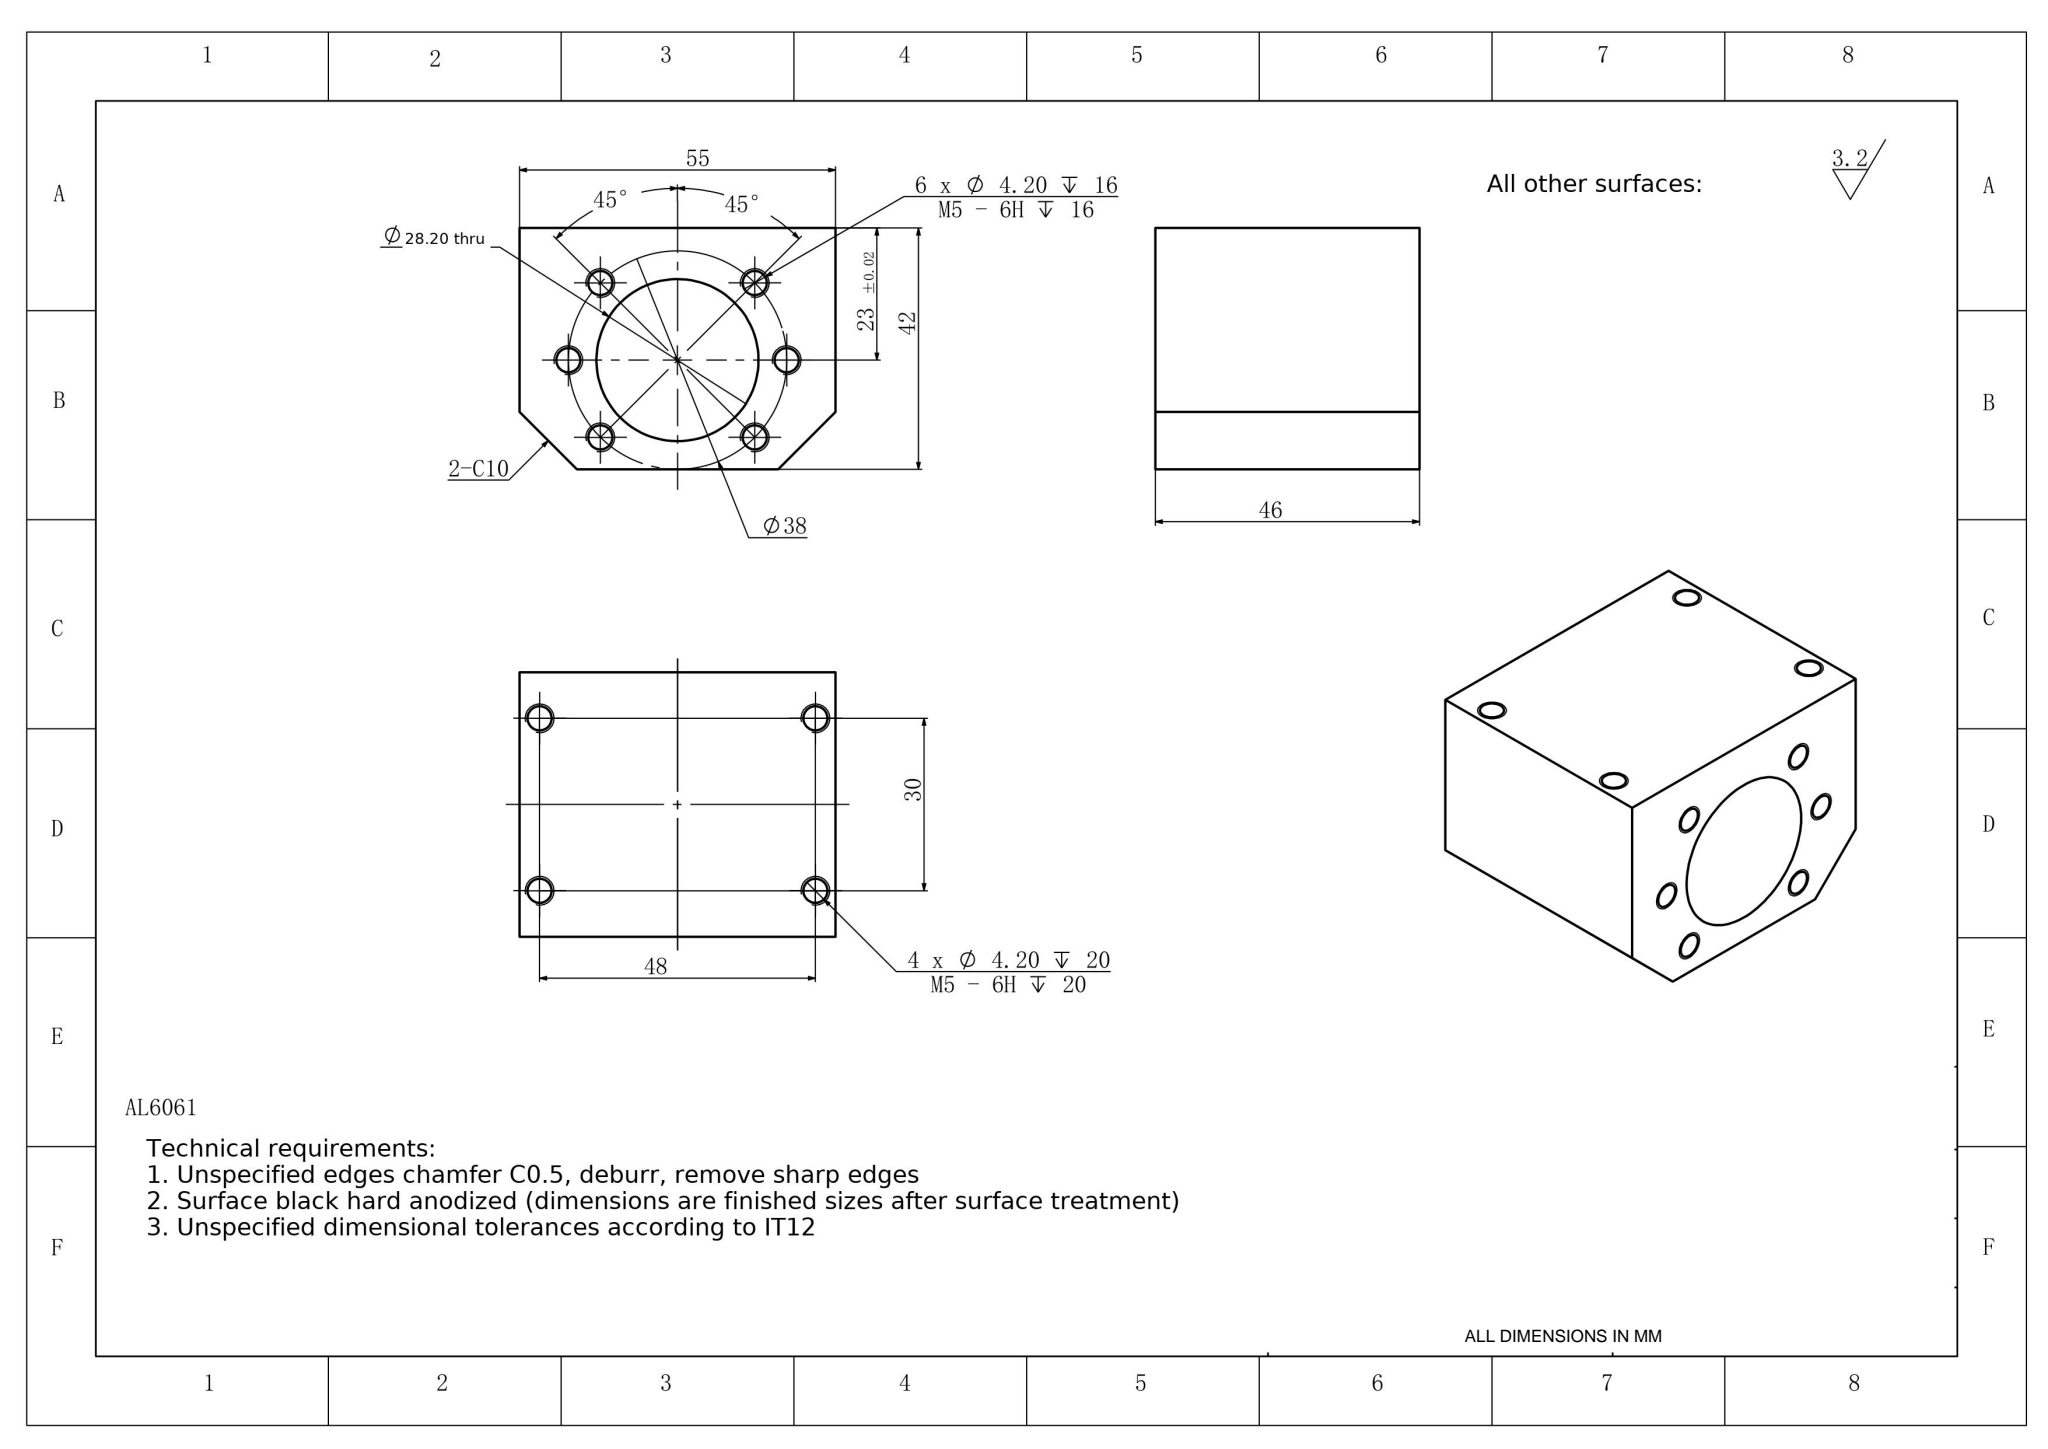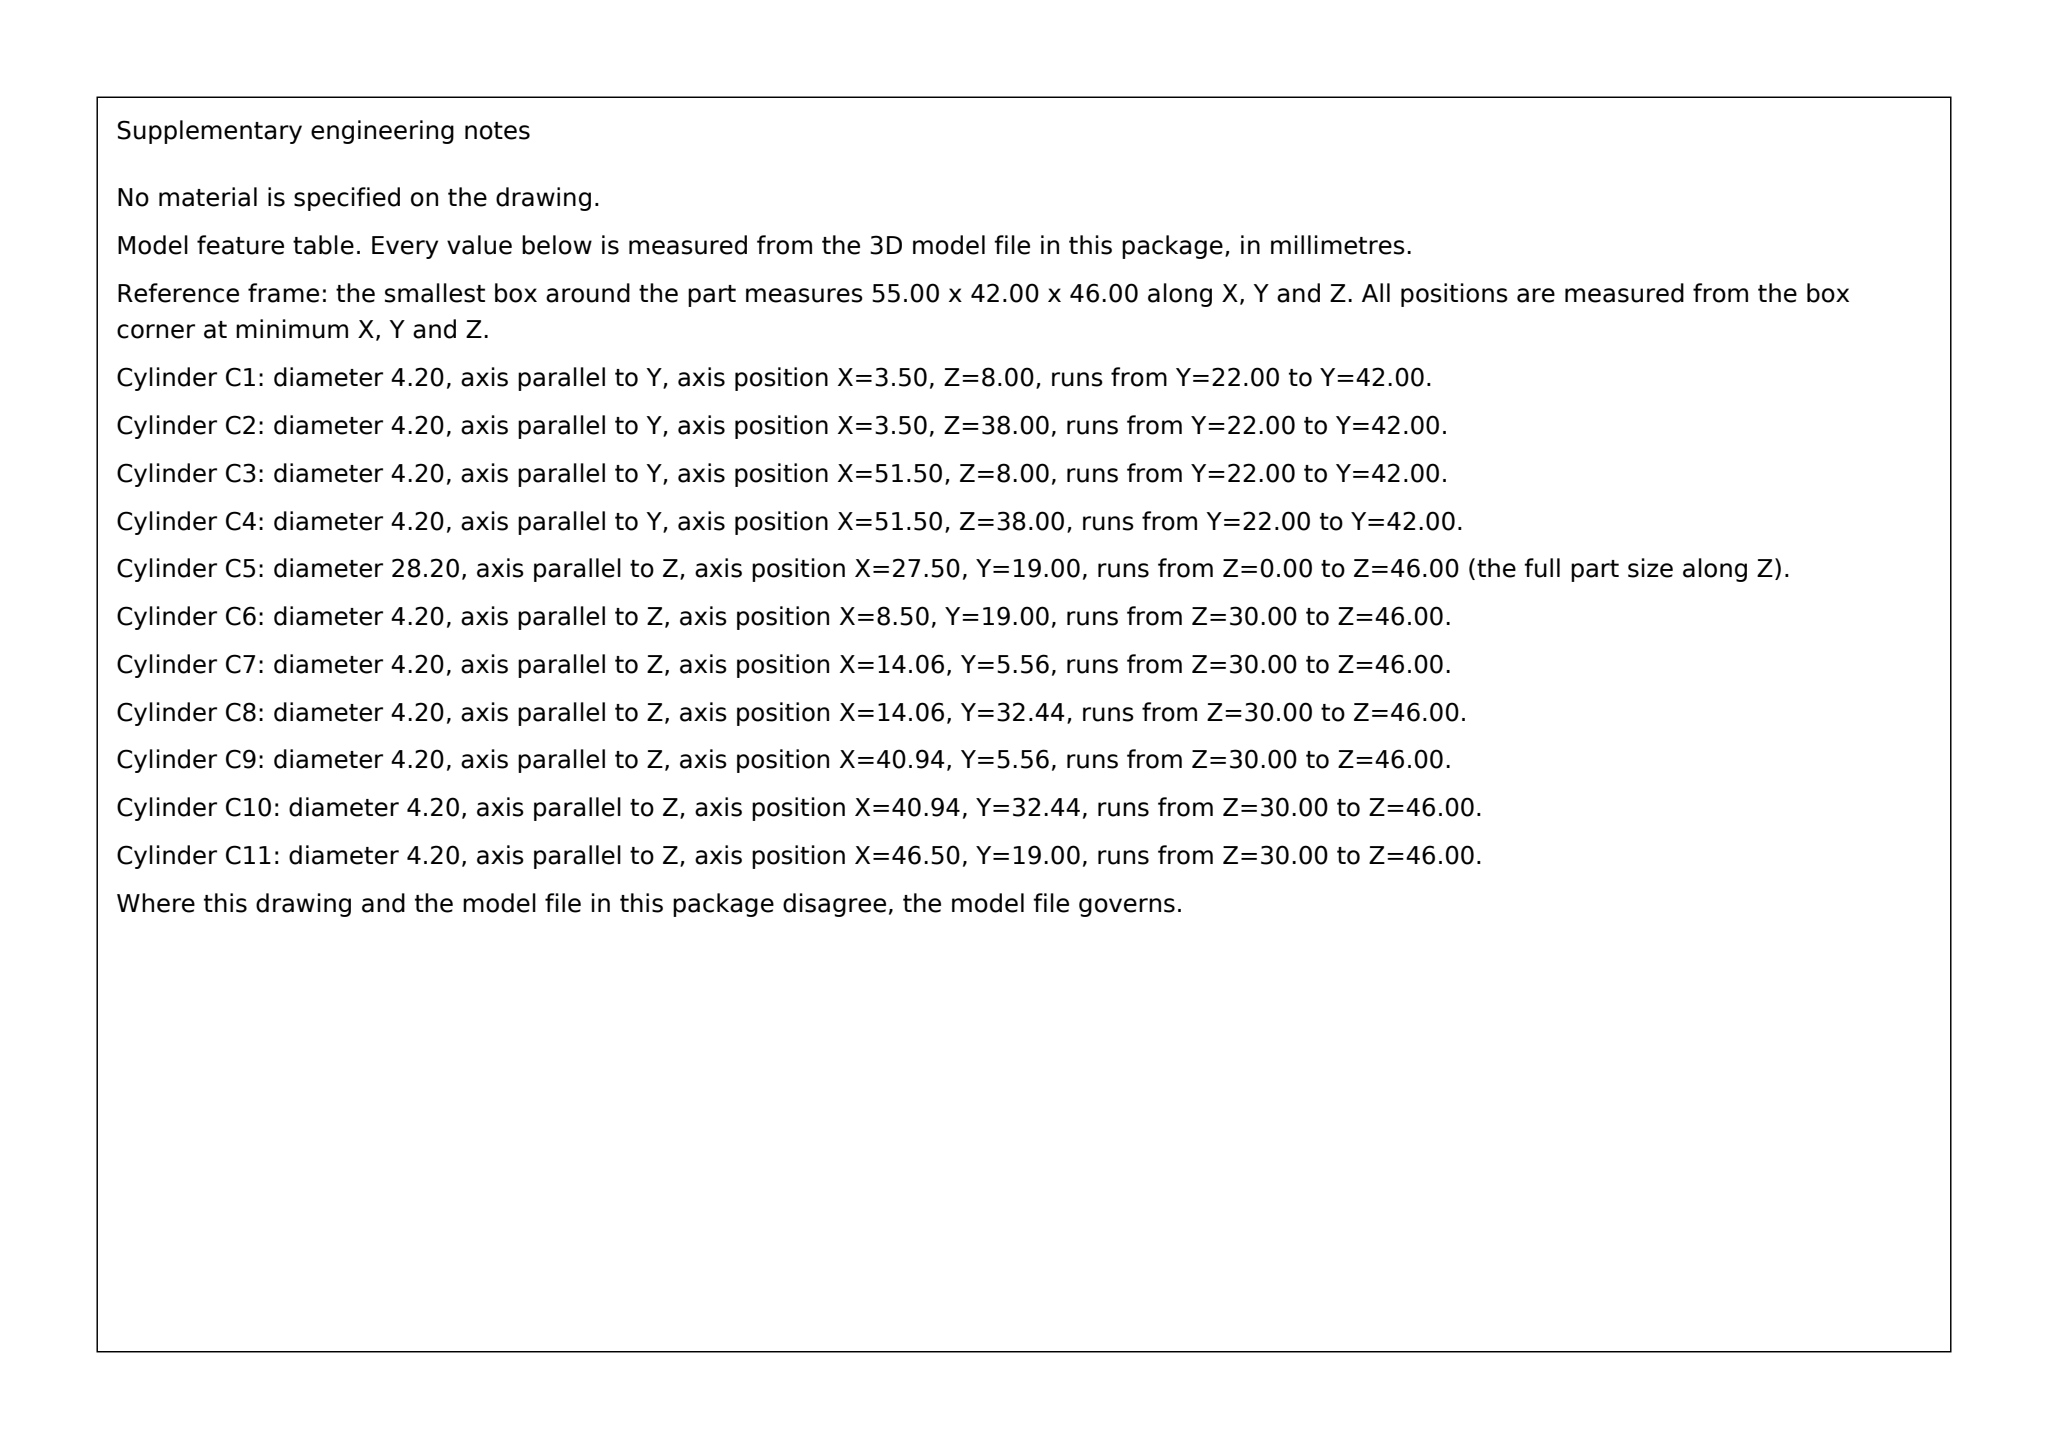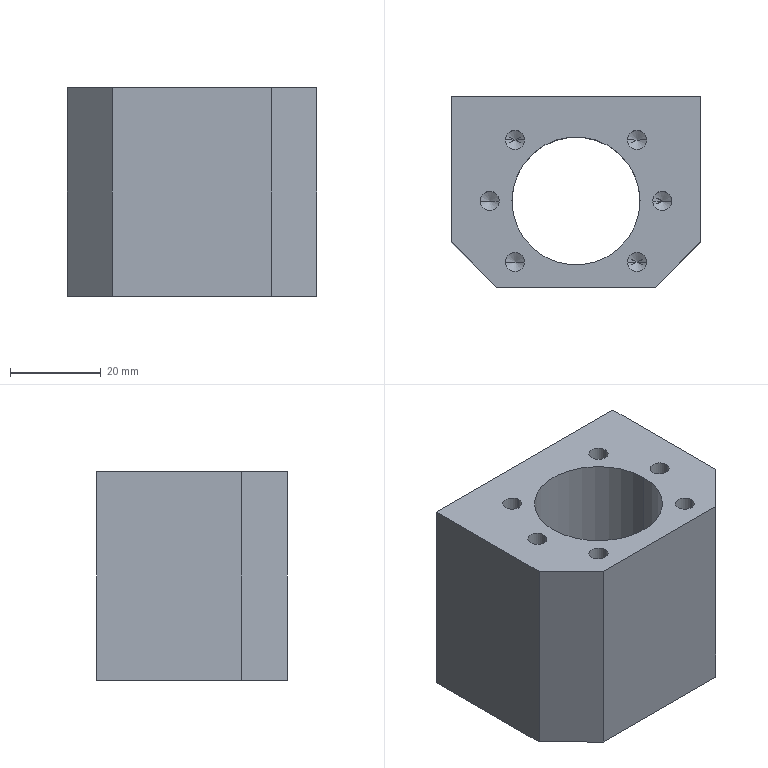Part | SolidWorks | mm | material AL6061 | 1 solid | 50 faces | box 55 x 42 x 46 mm | volume 70433 mm3 | cylinder 22 | cone 20 | plane 8 | commonest cylinder face diameters 4.2 x20 28.2 x2
build123d program:
from build123d import *

# Parameters (mm, degrees)
SKETCH1_W             = 55
SKETCH1_H             = 42
SKETCH1_R             = 14.1
EXTRUDE1_DEPTH        = 46
M5_TAPPED_HOLE3_D     = 4.2
M5_TAPPED_HOLE3_DEPTH = 16
M5_TAPPED_HOLE3_TIP   = 1.262
M5_TAPPED_HOLE4_D     = 4.2
M5_TAPPED_HOLE4_DEPTH = 20
M5_TAPPED_HOLE4_TIP   = 1.262
CHAMFER1_SIZE         = 10


with BuildPart() as part:
    # Sketch1 → Extrude1 (new body)
    with BuildSketch(Plane.XY):
        with Locations((27.5, 21)):
            Rectangle(SKETCH1_W, SKETCH1_H)
        with Locations((27.5, 19)):
            Circle(SKETCH1_R, mode=Mode.SUBTRACT)
    extrude(amount=EXTRUDE1_DEPTH)

    # M5 Tapped Hole3
    with Locations(Plane.XY.offset(46)):
        with Locations((14.065, 32.435), (8.5, 19), (14.065, 5.565), (40.935, 32.435), (46.5, 19), (40.935, 5.565)):
            Hole(M5_TAPPED_HOLE3_D / 2, depth=M5_TAPPED_HOLE3_DEPTH)
            with Locations((0, 0, -(M5_TAPPED_HOLE3_DEPTH + M5_TAPPED_HOLE3_TIP / 2))):  # 118° drill point
                Cone(0, M5_TAPPED_HOLE3_D / 2, M5_TAPPED_HOLE3_TIP, mode=Mode.SUBTRACT)

    # M5 Tapped Hole4
    with Locations(Plane(origin=(0, 42, 0), x_dir=(1, 0, 0), z_dir=(0, 1, 0))):
        with Locations((3.5, -8), (51.5, -8), (3.5, -38), (51.5, -38)):
            Hole(M5_TAPPED_HOLE4_D / 2, depth=M5_TAPPED_HOLE4_DEPTH)
            with Locations((0, 0, -(M5_TAPPED_HOLE4_DEPTH + M5_TAPPED_HOLE4_TIP / 2))):  # 118° drill point
                Cone(0, M5_TAPPED_HOLE4_D / 2, M5_TAPPED_HOLE4_TIP, mode=Mode.SUBTRACT)

    # Chamfer1
    chamfer1_edges = [part.edges().sort_by_distance(p)[0] for p in [
        (55, 0, 23),
        (0, 0, 23),
    ]]
    chamfer(chamfer1_edges, length=CHAMFER1_SIZE)


solid = part.part